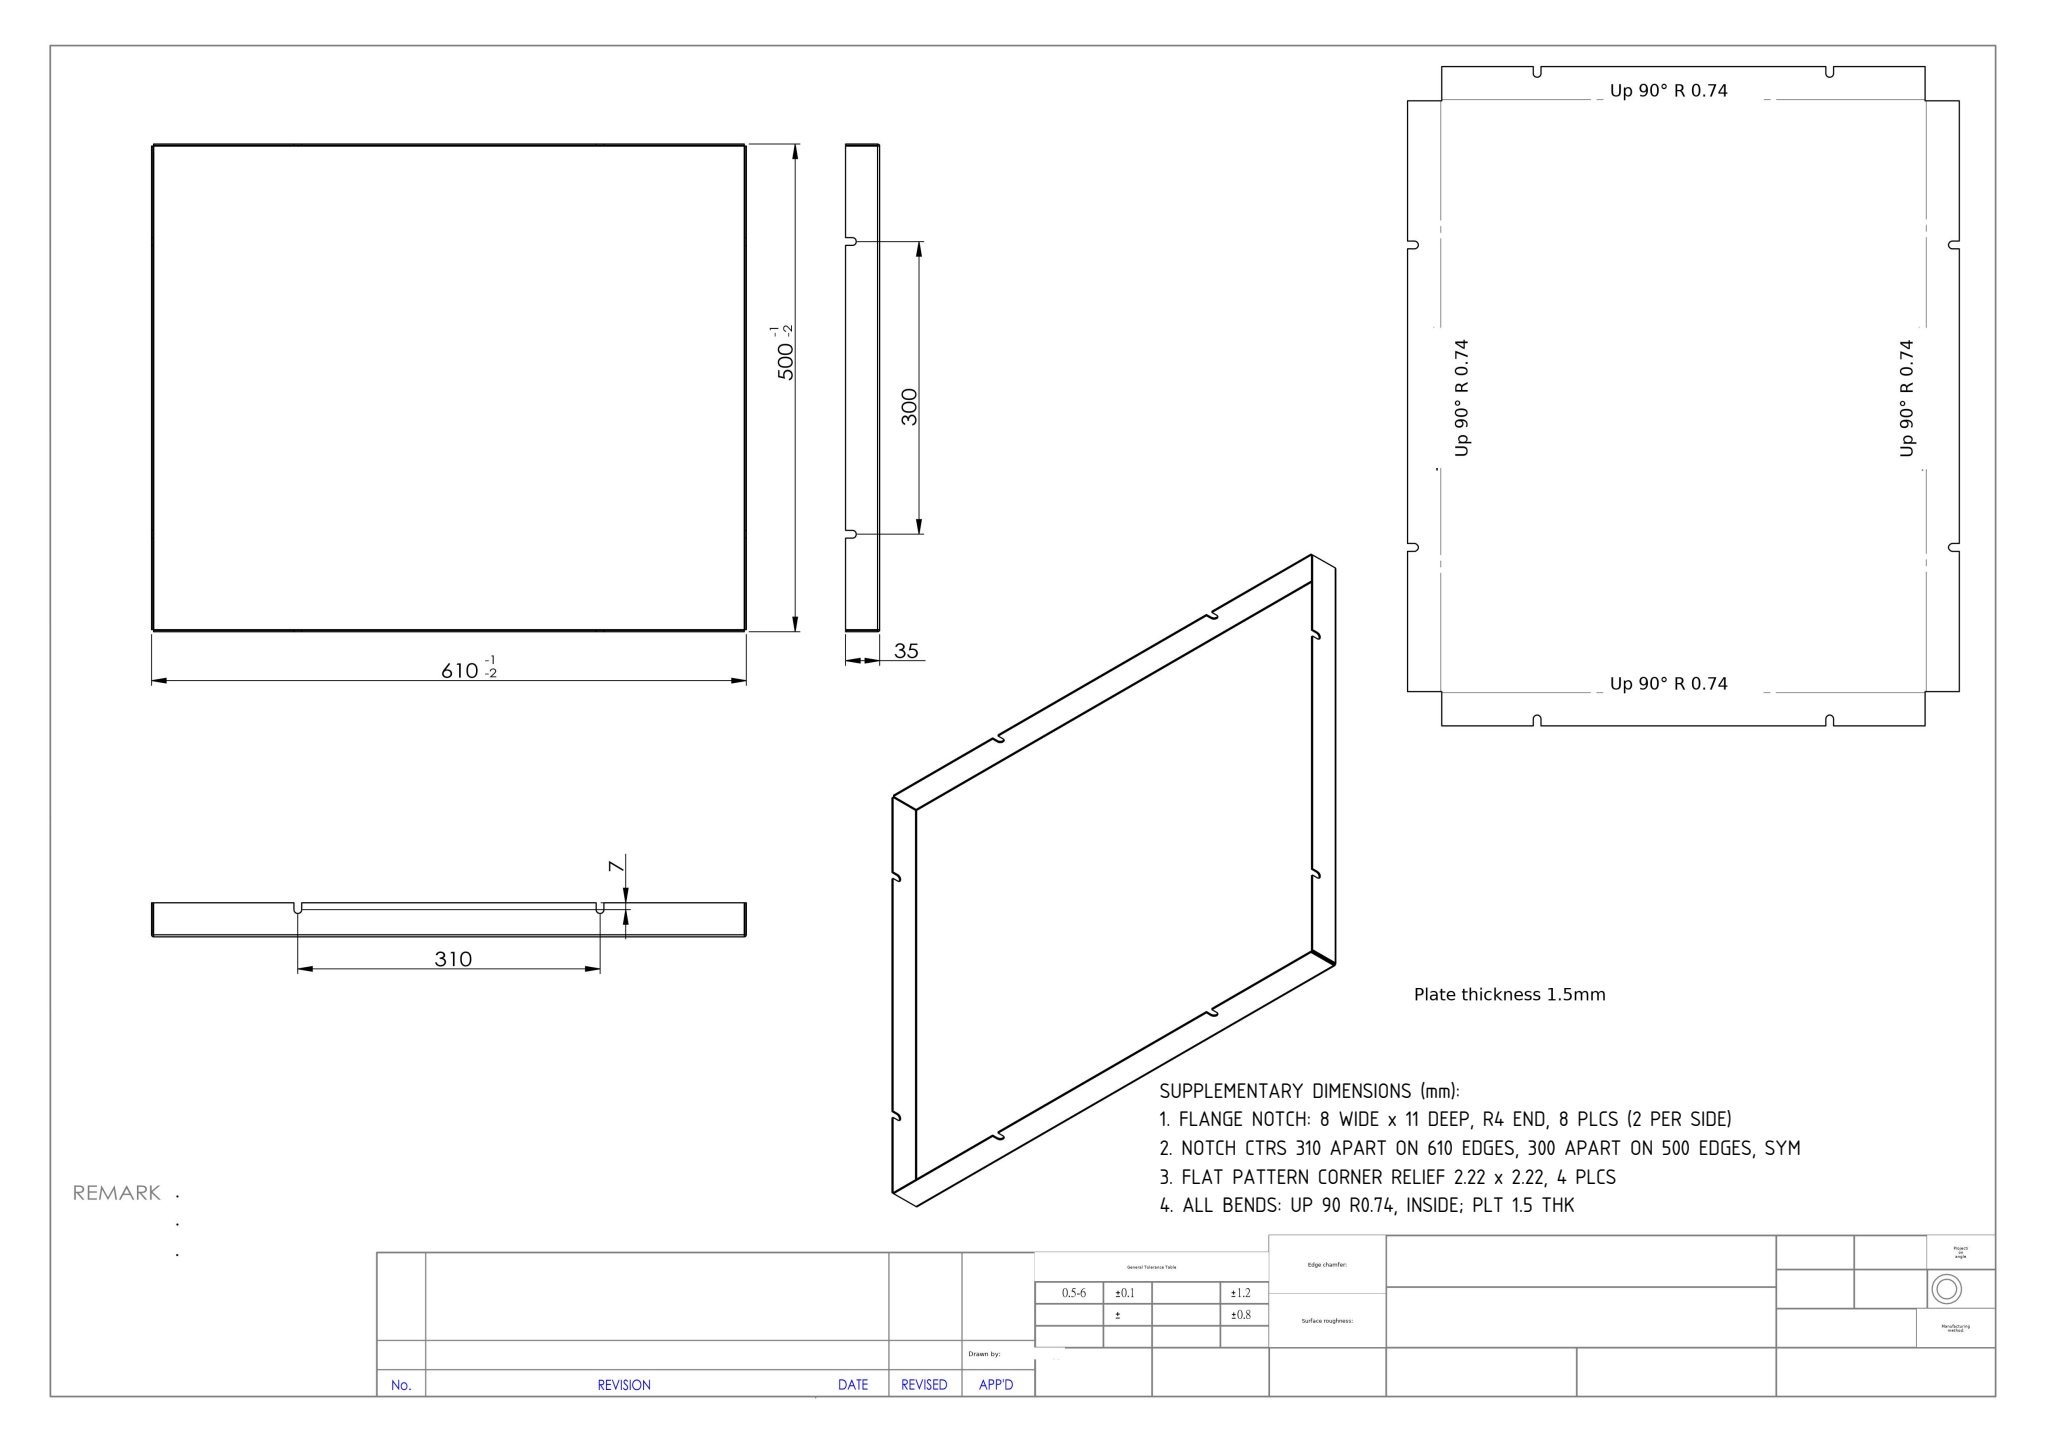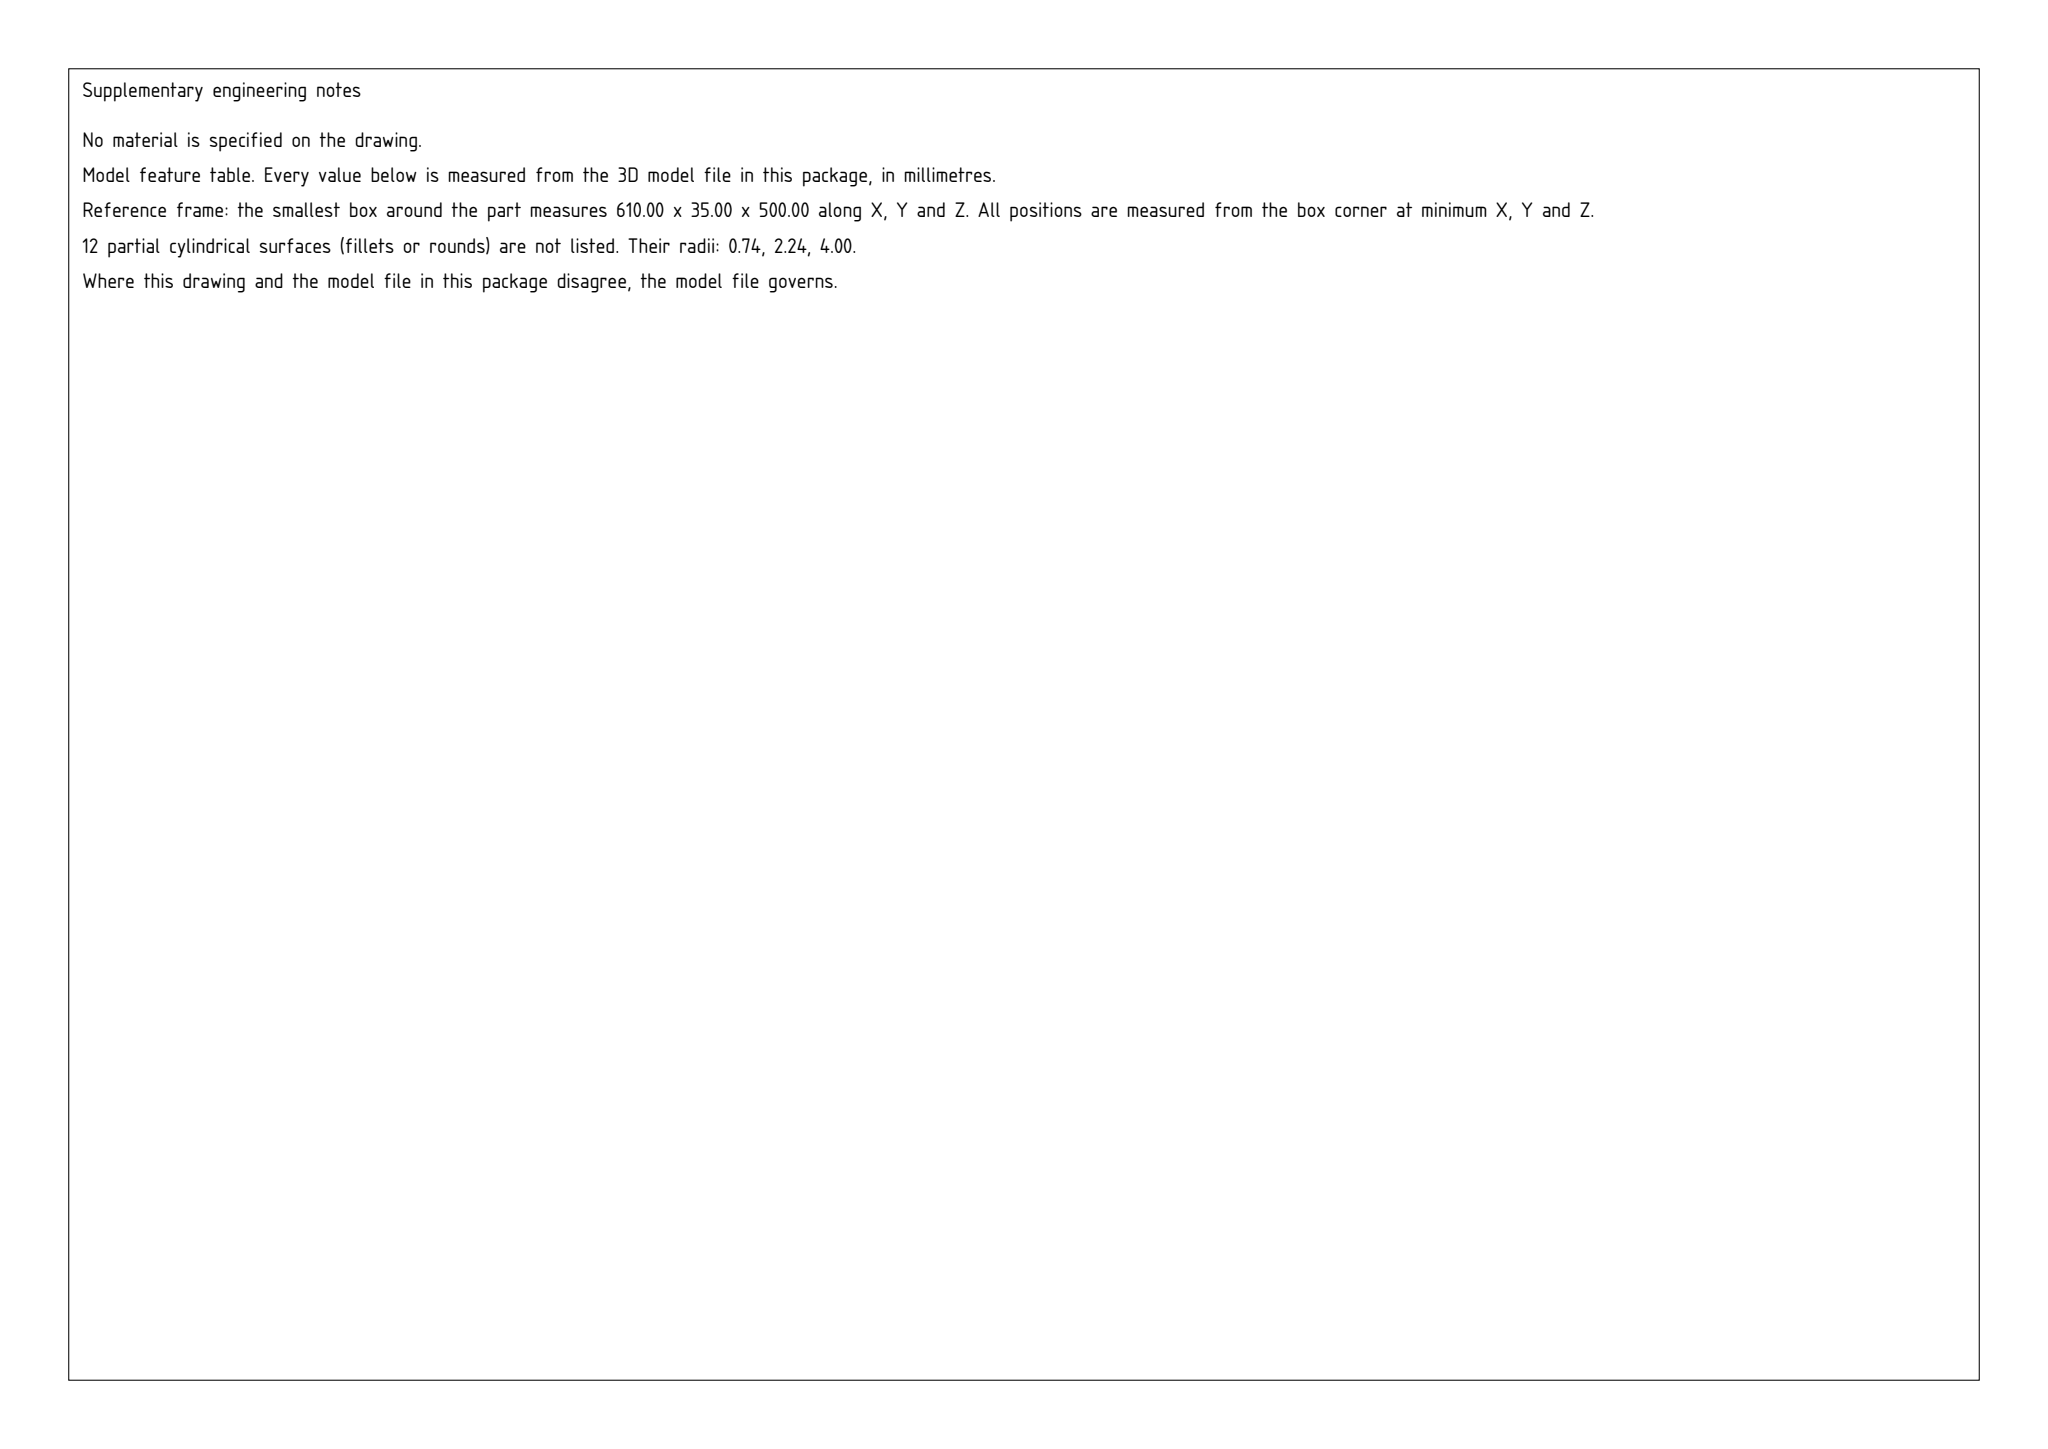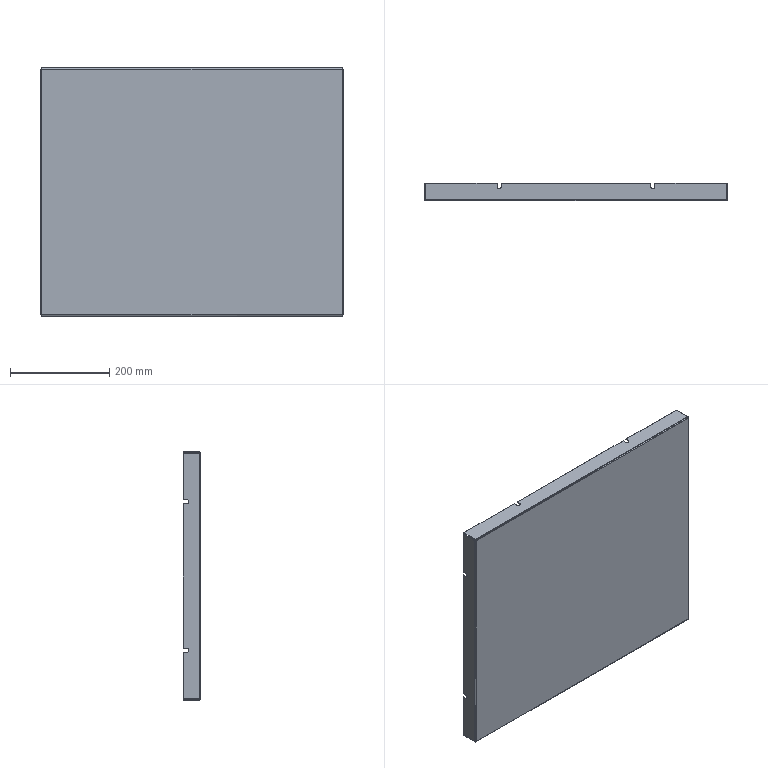Part | SolidWorks | mm | 1 solid | 74 faces | box 610 x 35 x 500 mm | volume 565057 mm3 | plane 46 | cylinder 20 | spline 8 | commonest cylinder face diameters 8 x12 4.473 x4 1.473 x4